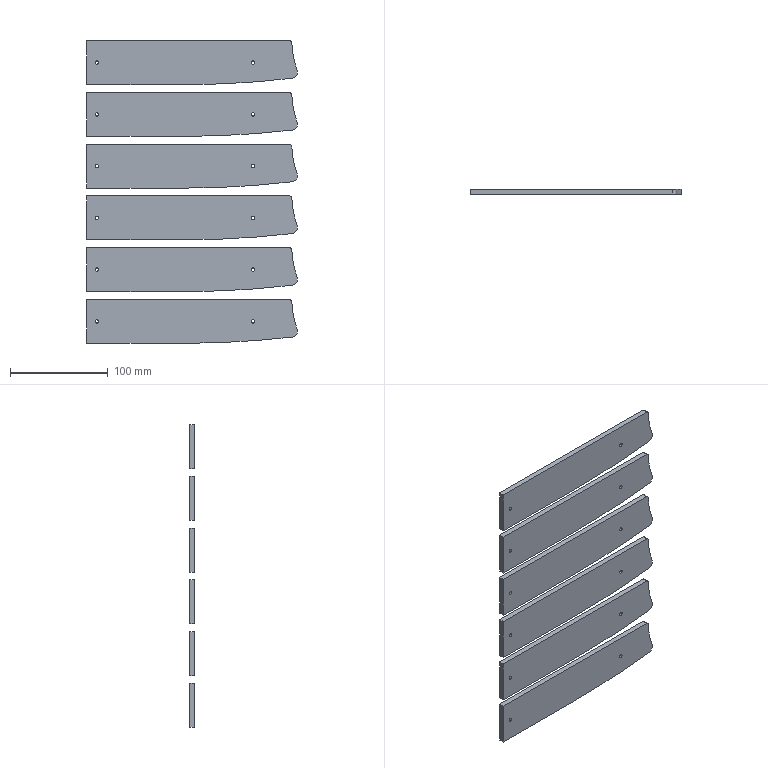CAM job | Mastercam | mm | 4 operations | part box 215.94 x 5 x 310
1. Contour (Ramp) | 3 - 3 平铣刀
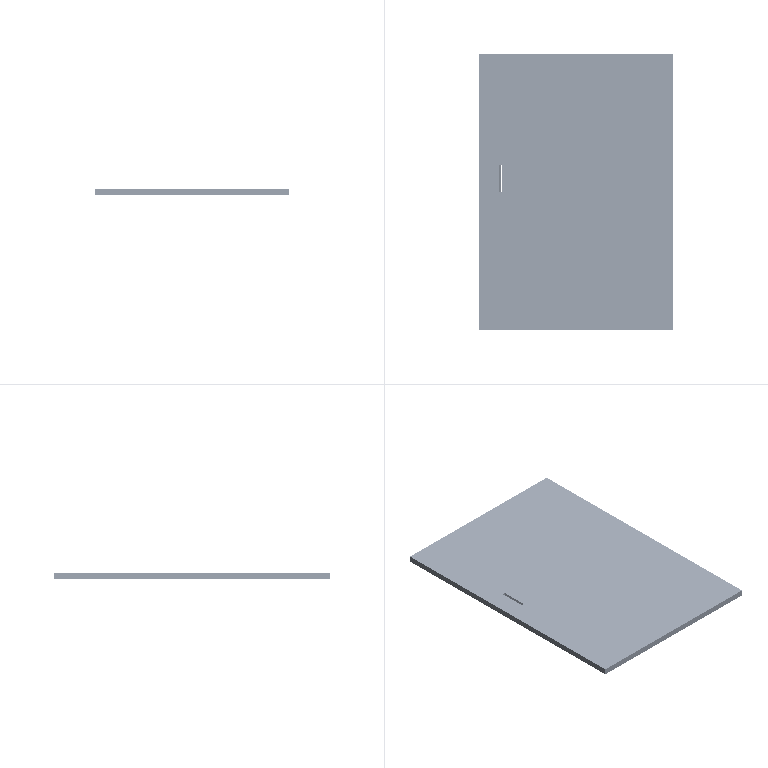2. Contour (2D chamfer) | 7 - 4 倒角刀
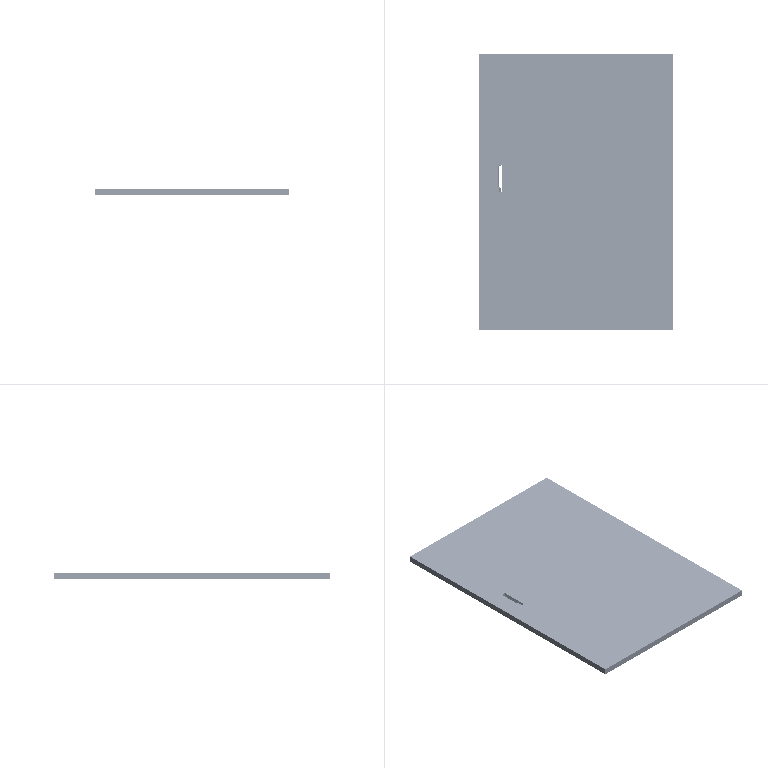3. Drill/Counterbore | 7 - 4 倒角刀
4. Contour (Ramp) | 2 - 2 平铣刀